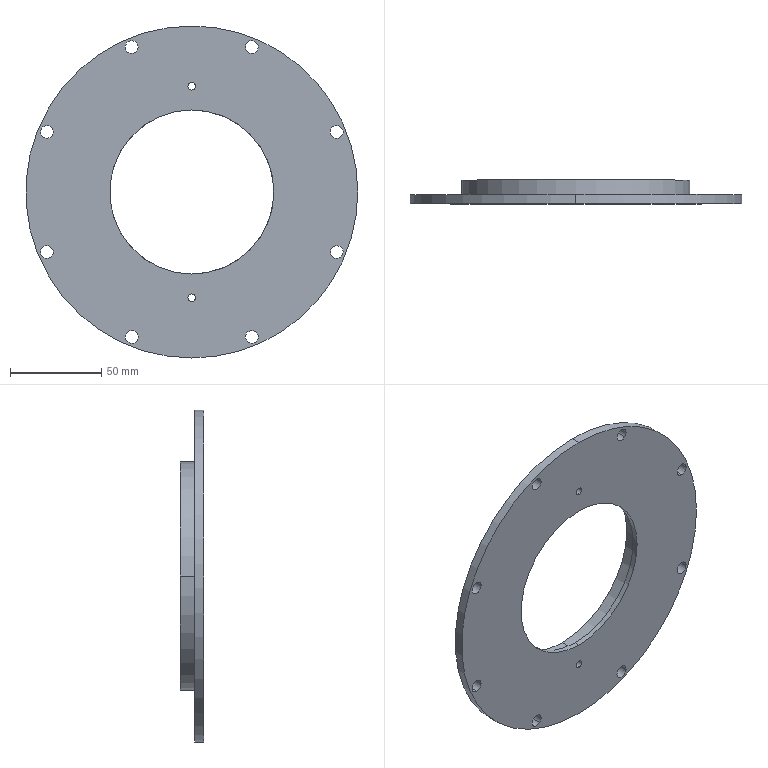CAM job | Mastercam | mm | 10 operations | part box 182 x 13 x 182
1. Facing | 24 - 100 平铣刀
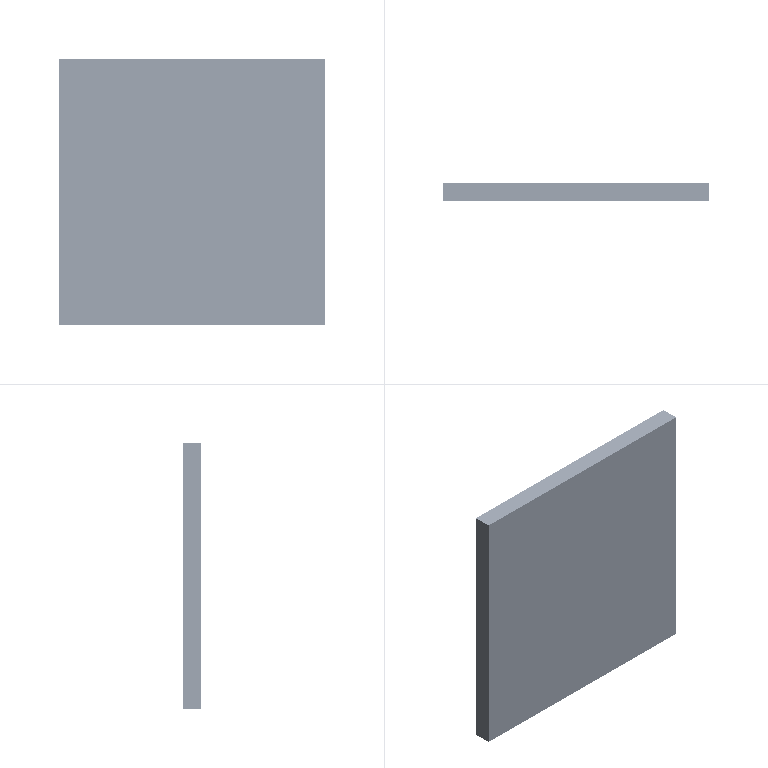2. 2D High Speed (2D Area Mill) | 9 - 10 平铣刀
3. Contour (Ramp) | 9 - 10 平铣刀
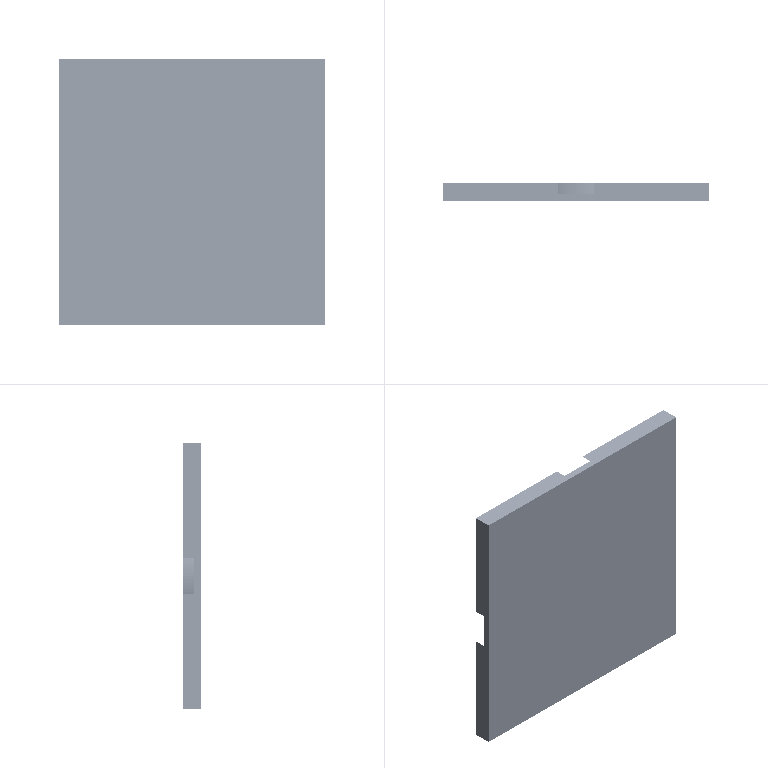4. 2D High Speed (2D Area Mill) | 10 - 10 平铣刀
5. Contour (2D) | 10 - 10 平铣刀
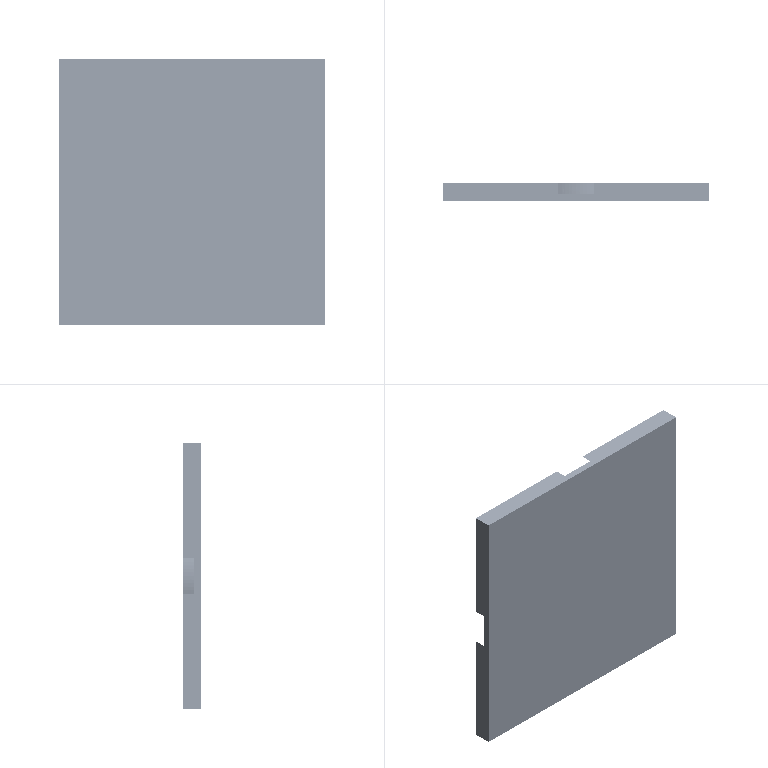6. Contour (2D) | 10 - 10 平铣刀
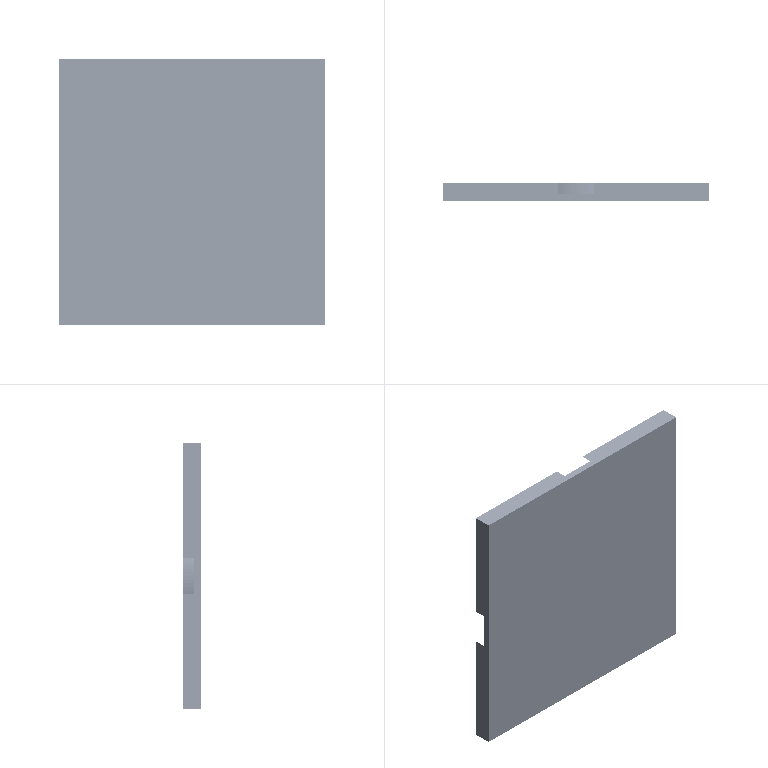7. Contour (Ramp) | 4 - 4 平铣刀
8. Contour (2D chamfer) | 5 - 4 倒角刀
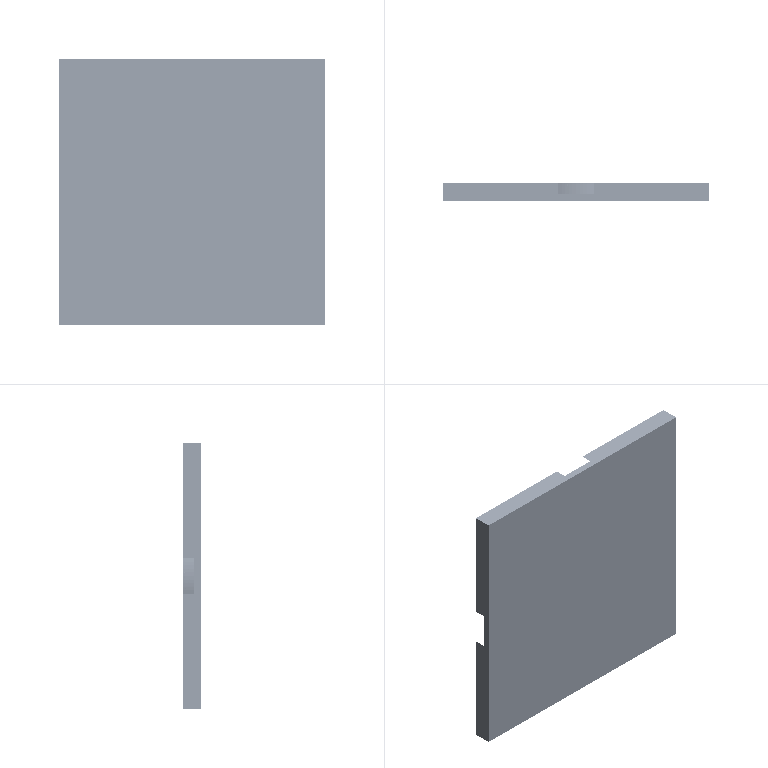9. Drill/Counterbore | 5 - 4 倒角刀
10. Contour (2D) | 3 - 3 平铣刀